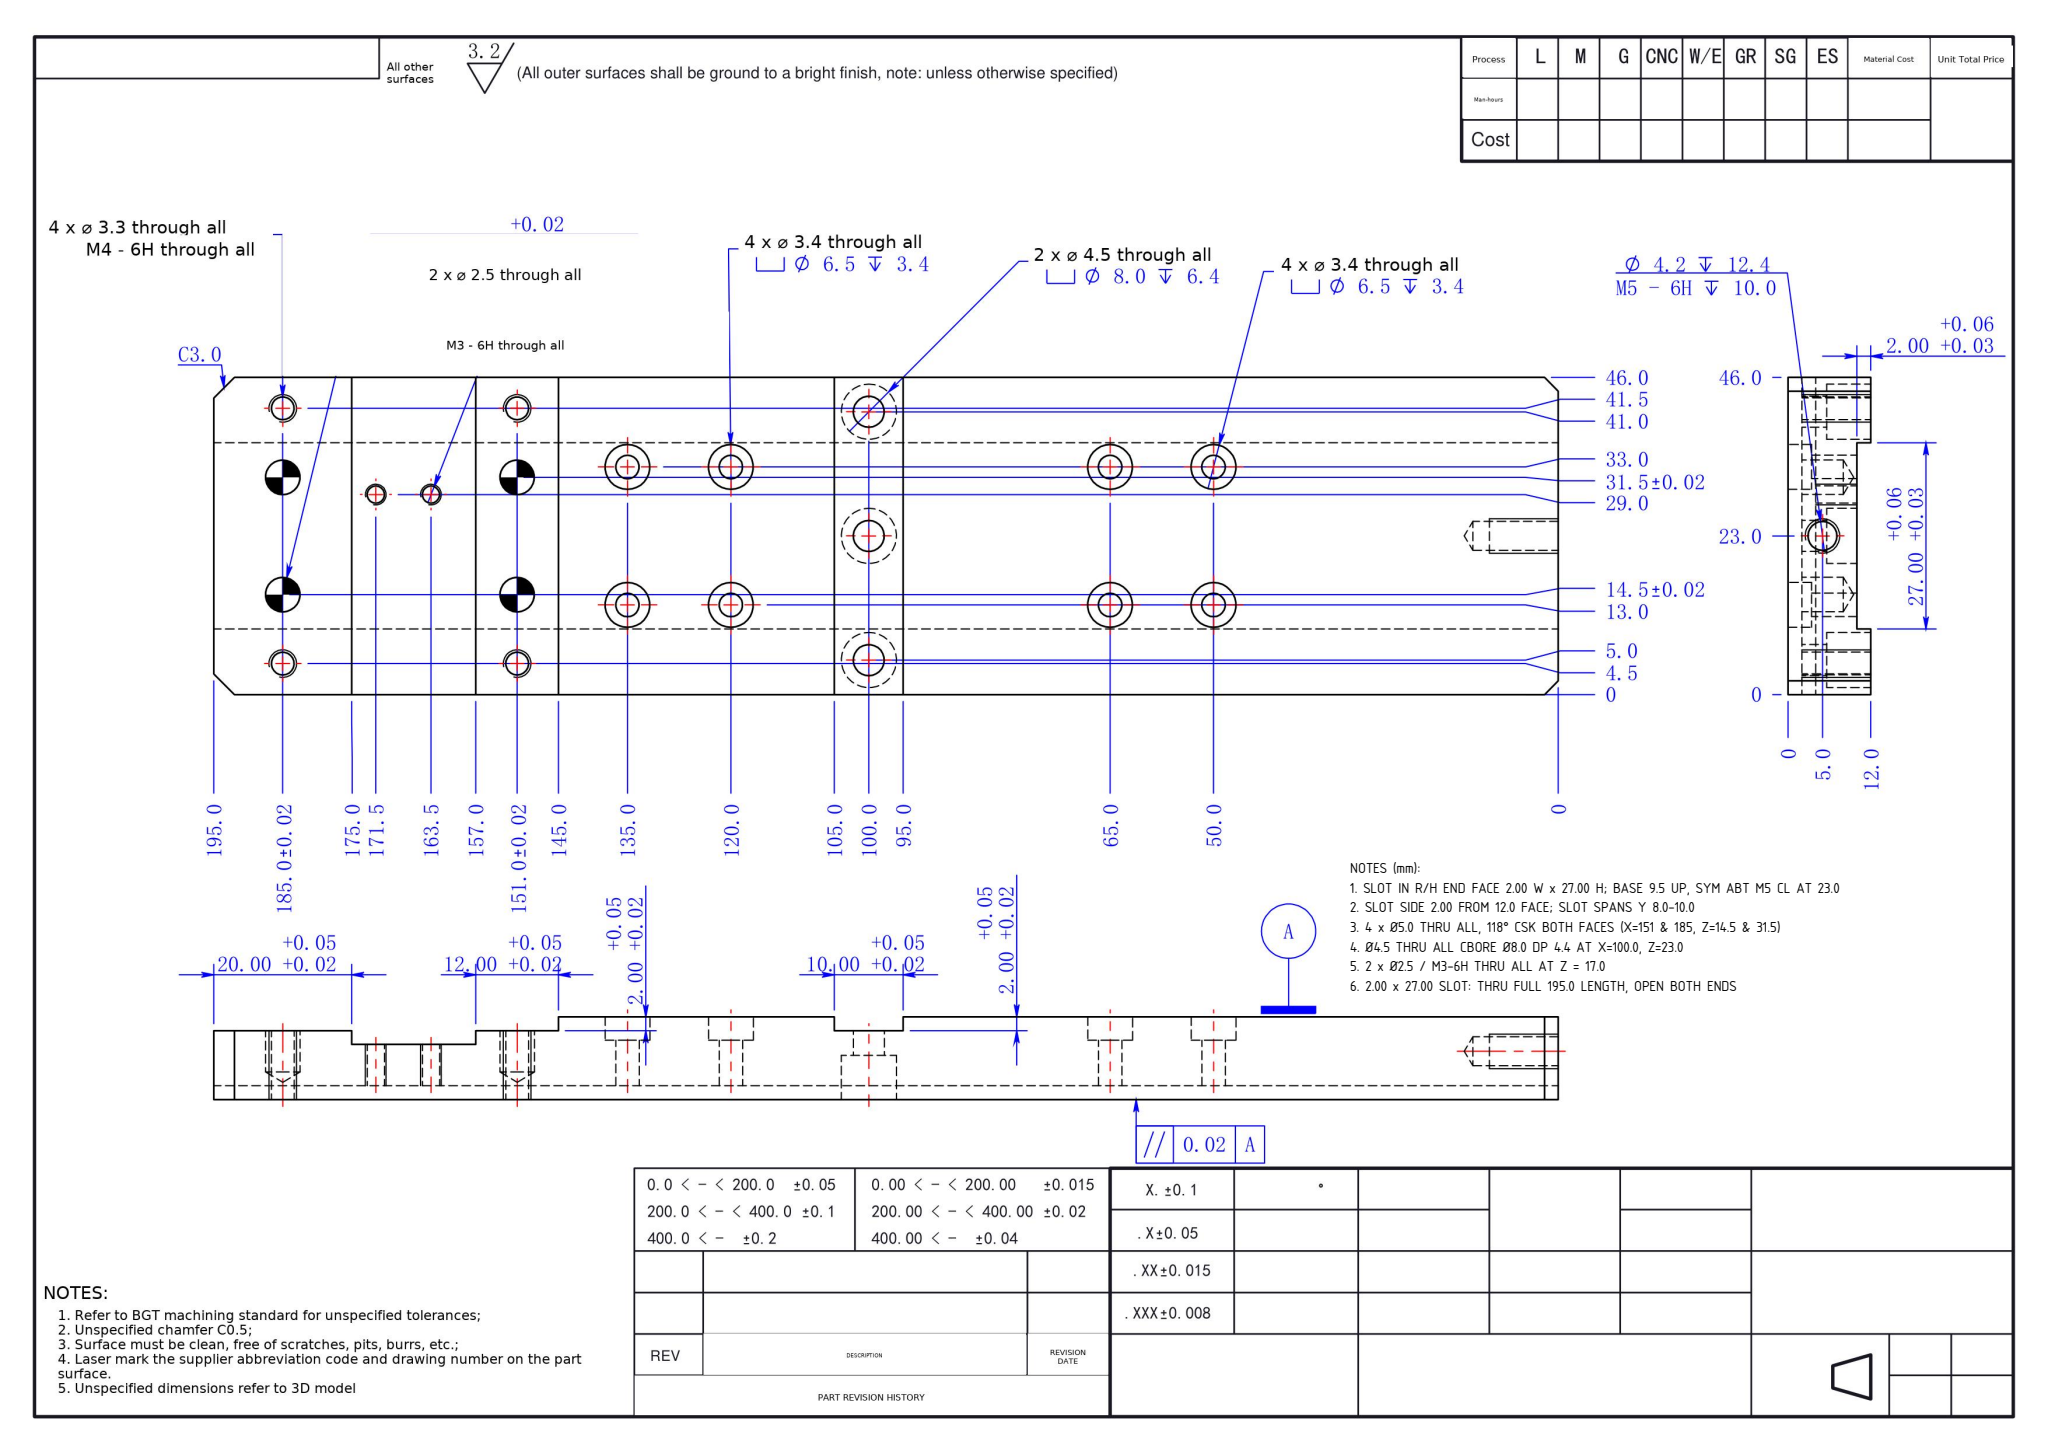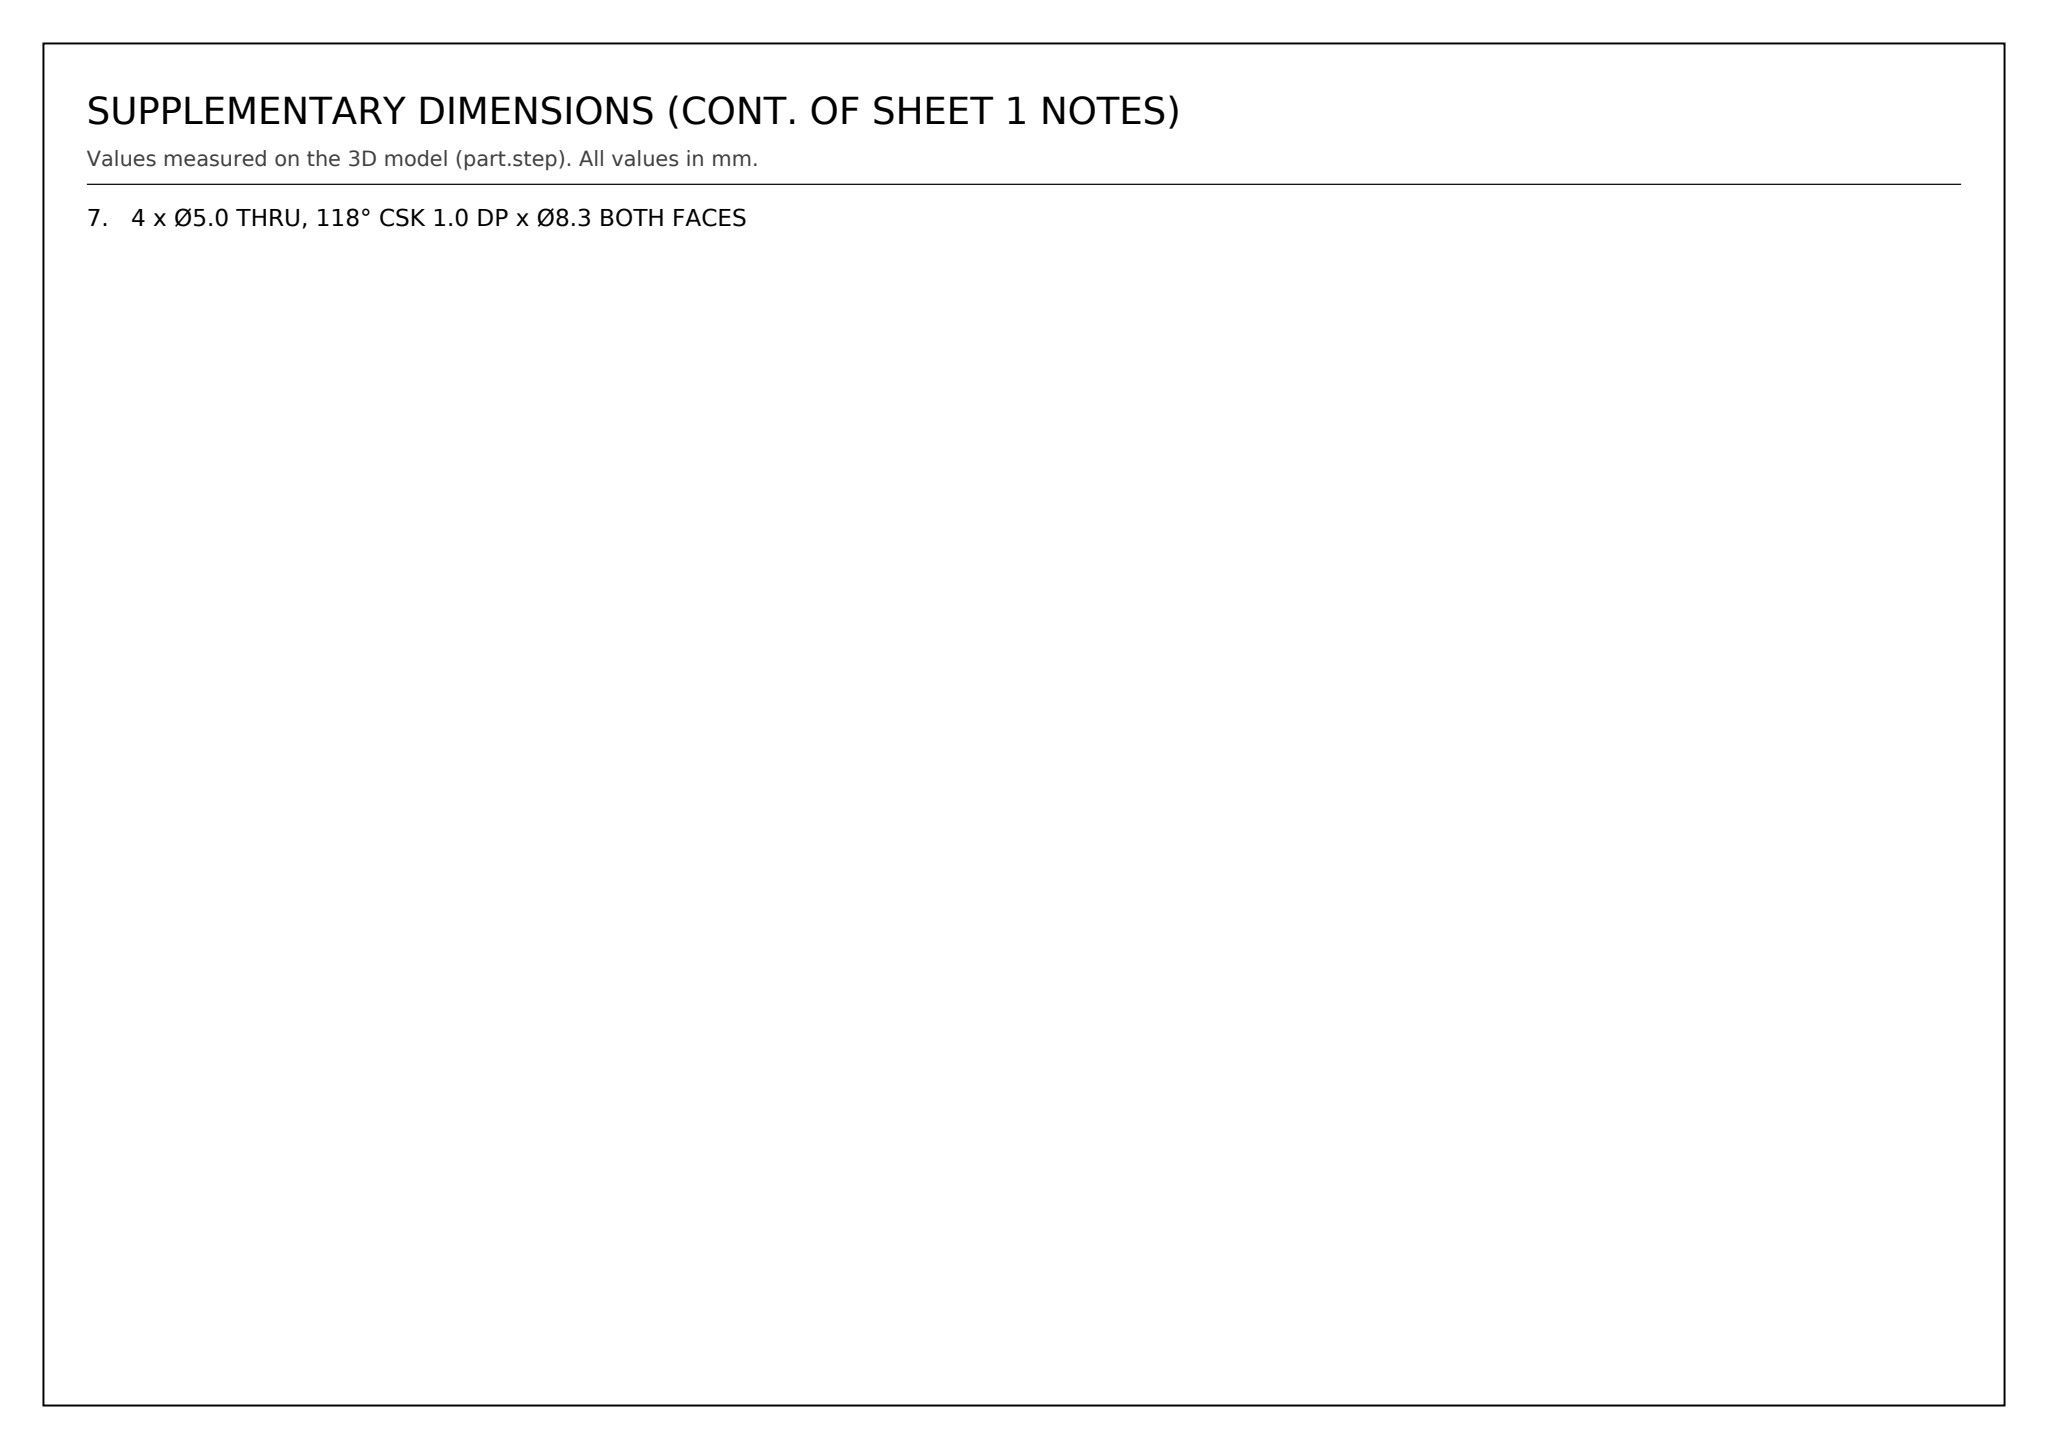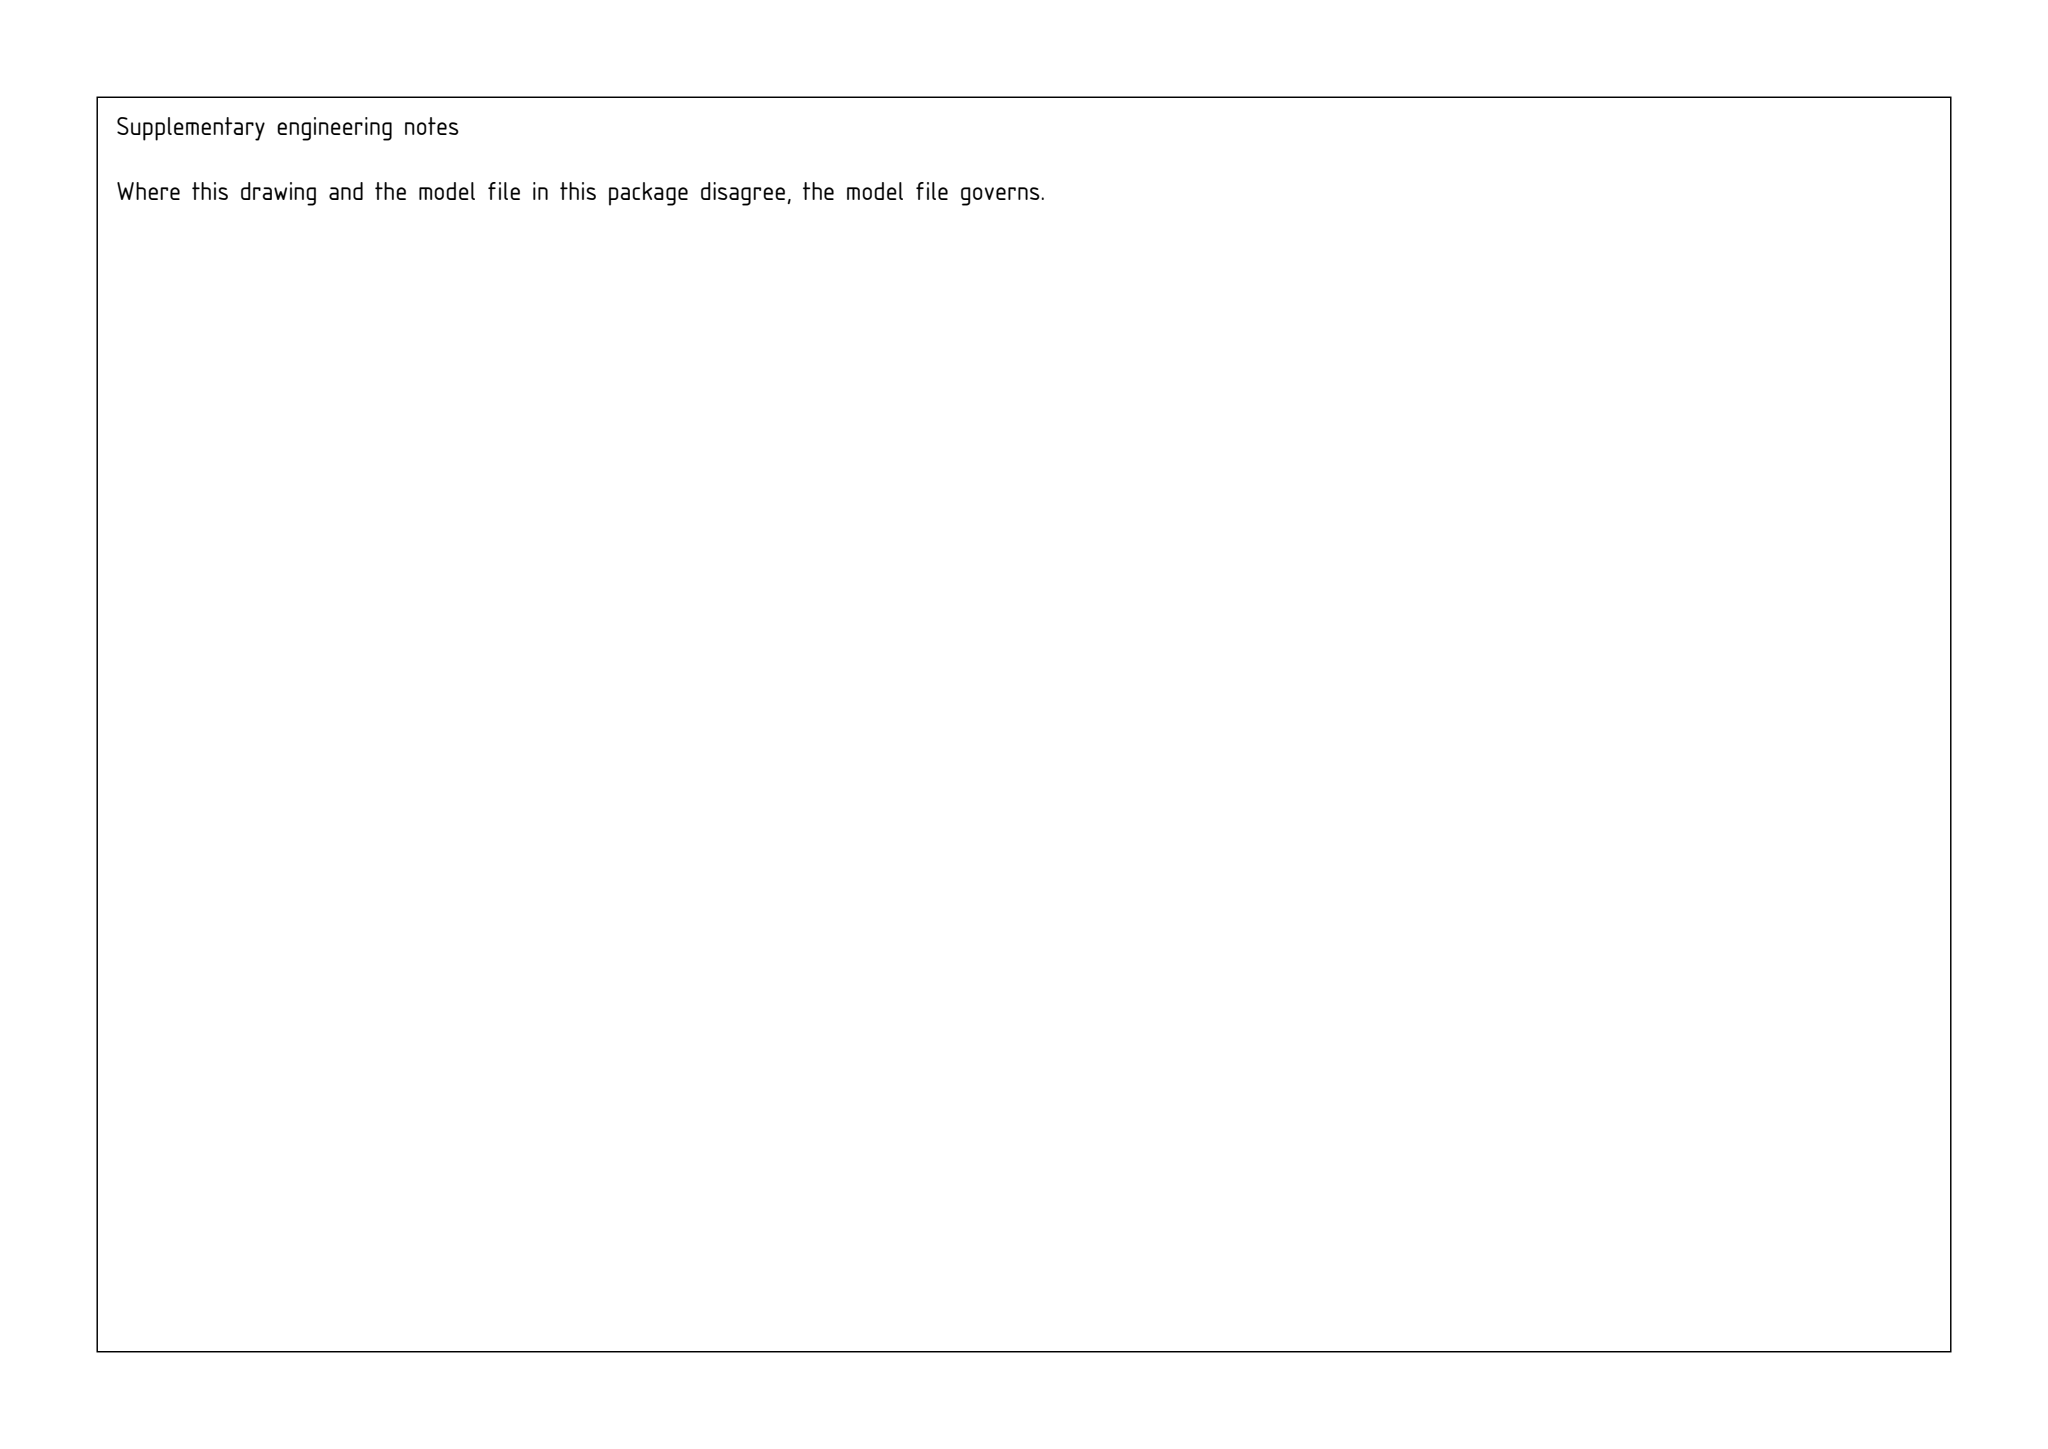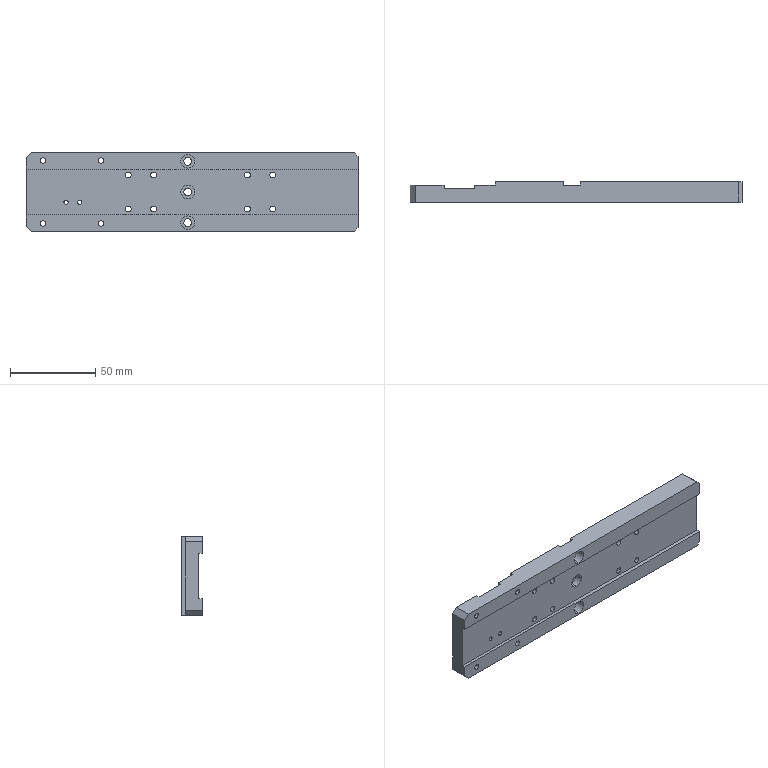Part | SolidWorks | mm | 1 solid | 111 faces | box 195 x 12 x 46 mm | volume 86288 mm3 | cylinder 66 | plane 35 | cone 10 | commonest cylinder face diameters 6.5 x16 3.4 x16 5 x8 3.3 x8 8 x6 4.5 x6 2.5 x4 4.2 x2
Drawing notes:
SLOT IN R/H END FACE 2.00 W x 27.00 H; BASE 9.5 UP, SYM ABT M5 CL AT 23.0 | from the solid: y walls 8.0 & 10.0 = 2.0 wide; z walls 9.5 & 36.5 = 27.0 high, CL 23.0; Ø4.2 x-axis hole at z=23.0
SLOT SIDE 2.00 FROM 12.0 FACE; SLOT SPANS Y 8.0-10.0 | from the solid: y plane 10.0 vs part face y=12.0 (bbox y=12.0); slot y 8.0-10.0
4 x Ø5.0 THRU ALL, 118° CSK BOTH FACES (X=151 & 185, Z=14.5 & 31.5) | from the solid: cyl Ø5.0 axis y at (10,14.5),(10,31.5),(44,14.5),(44,31.5) L=6.0 each side; cones 118° ref dia 5.0, qty 8
Ø4.5 THRU ALL CBORE Ø8.0 DP 4.4 AT X=100.0, Z=23.0 | from the solid: cyl Ø4.5 axis y at x=95 (=195-95=100 ord), z=23.0; c'bore Ø8.0 depth 4.4
2 x Ø2.5 / M3-6H THRU ALL AT Z = 17.0 | from the solid: cyl Ø2.5 axis y at z=17.0, x=23.5 & 31.5 (ord 171.5 & 163.5)
2.00 x 27.00 SLOT: THRU FULL 195.0 LENGTH, OPEN BOTH ENDS | from the solid: Slot bounded by y=0-2.00 and z=9.50-36.50 (27.00); no x-normal end face between x=0 and x=195 - Ø6.5 CB holes at x=60/145 give 3.4 cyl len 6.6 (8.6-2.0) and Ø8 CB at x=95,z=23 len 4.4 (6.4-2.0), proving slot present over full length
4 x Ø5.0 THRU, 118° CSK 1.0 DP x Ø8.3 BOTH FACES | from the solid: cones[118.0,5.0]x8 = 2 per hole on 4 x Ø5.0 holes; Ø5.0 cyl len 6.0 in 8.0 wall (y=2.0 to 10.0) -> 1.0 csk each face; 5.0+2x1.0xtan59°=8.33